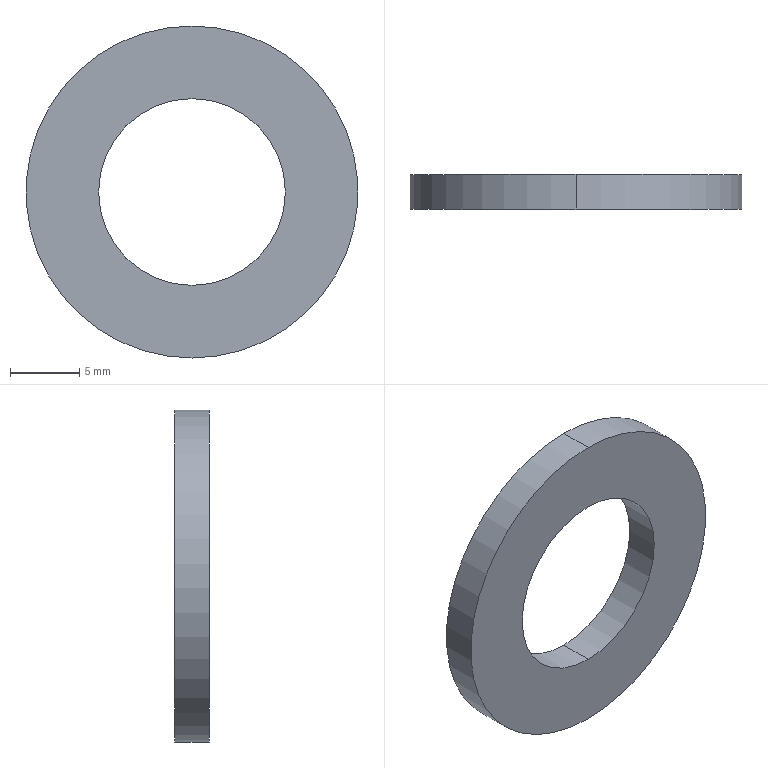Component | SolidWorks | GB_T95-2002[FlatWasherC-grade12]-1 | 1 solid | 6 faces | box 24 x 2.5 x 24 mm | volume 773 mm3 | cylinder 4 | plane 2 | commonest cylinder face diameters 24 x2 13.5 x2
build123d program:
from build123d import *

# Parameters (mm, degrees)
SKETCH1_W = 5.25
SKETCH1_H = 2.5


with BuildPart() as part:
    # Sketch1 → Base-Revolve (revolve)
    with BuildSketch(Plane.XY, mode=Mode.PRIVATE) as base_revolve_sk:
        with Locations((-9.375, 9.895)):
            Rectangle(SKETCH1_W, SKETCH1_H)
    revolve(base_revolve_sk.sketch.rotate(Axis((0, 0, 0), (0, 1, 0)), 270), axis=Axis((0, 0, 0), (0, 1, 0)))


solid = part.part

# Placed as in the assembly
solid = solid.moved(Location((96, 205.461, 0), (0, 0, 0)))
STEP:
#1=COLOUR_RGB('',0.7922,0.8196,0.9333);
#2=FILL_AREA_STYLE_COLOUR('',#1);
#3=FILL_AREA_STYLE('',(#2));
#4=SURFACE_STYLE_FILL_AREA(#3);
#5=SURFACE_SIDE_STYLE('',(#4));
#6=SURFACE_STYLE_USAGE(.BOTH.,#5);
#7=PRESENTATION_STYLE_ASSIGNMENT((#6));
#8=CARTESIAN_POINT('',(3.78,8.528,-0.4724));
#9=VERTEX_POINT('',#8);
#10=CARTESIAN_POINT('',(3.78,8.528,0.4724));
#11=VERTEX_POINT('',#10);
#12=CARTESIAN_POINT('',(3.78,8.528,0.));
#13=DIRECTION('',(0.,-1.,0.));
#14=DIRECTION('',(0.,0.,-1.));
#15=AXIS2_PLACEMENT_3D('',#12,#13,#14);
#16=CIRCLE('',#15,0.4724);
#17=EDGE_CURVE('',#9,#11,#16,.T.);
#18=ORIENTED_EDGE('',*,*,#17,.T.);
#19=CARTESIAN_POINT('',(3.78,8.429,0.4724));
#20=VERTEX_POINT('',#19);
#21=CARTESIAN_POINT('',(3.78,8.089,0.4724));
#22=DIRECTION('',(0.,-1.,0.));
#23=VECTOR('',#22,39.37);
#24=LINE('',#21,#23);
#25=EDGE_CURVE('',#11,#20,#24,.T.);
#26=ORIENTED_EDGE('',*,*,#25,.T.);
#27=CARTESIAN_POINT('',(3.78,8.429,-0.4724));
#28=VERTEX_POINT('',#27);
#29=CARTESIAN_POINT('',(3.78,8.429,0.));
#30=DIRECTION('',(0.,-1.,0.));
#31=DIRECTION('',(0.,0.,-1.));
#32=AXIS2_PLACEMENT_3D('',#29,#30,#31);
#33=CIRCLE('',#32,0.4724);
#34=EDGE_CURVE('',#28,#20,#33,.T.);
#35=ORIENTED_EDGE('',*,*,#34,.F.);
#36=CARTESIAN_POINT('',(3.78,8.089,-0.4724));
#37=DIRECTION('',(0.,-1.,0.));
#38=VECTOR('',#37,39.37);
#39=LINE('',#36,#38);
#40=EDGE_CURVE('',#9,#28,#39,.T.);
#41=ORIENTED_EDGE('',*,*,#40,.F.);
#42=EDGE_LOOP('',(#18,#26,#35,#41));
#43=FACE_OUTER_BOUND('',#42,.T.);
#44=CARTESIAN_POINT('',(3.78,8.089,0.));
#45=DIRECTION('',(0.,-1.,0.));
#46=DIRECTION('',(0.,0.,-1.));
#47=AXIS2_PLACEMENT_3D('',#44,#45,#46);
#48=CYLINDRICAL_SURFACE('',#47,0.4724);
#49=ADVANCED_FACE('',(#43),#48,.T.);
#50=CARTESIAN_POINT('',(3.78,8.528,0.2657));
#51=VERTEX_POINT('',#50);
#52=CARTESIAN_POINT('',(3.78,8.528,-0.2657));
#53=VERTEX_POINT('',#52);
#54=CARTESIAN_POINT('',(3.78,8.528,0.));
#55=DIRECTION('',(0.,-1.,0.));
#56=DIRECTION('',(0.,0.,-1.));
#57=AXIS2_PLACEMENT_3D('',#54,#55,#56);
#58=CIRCLE('',#57,0.2657);
#59=EDGE_CURVE('',#51,#53,#58,.T.);
#60=ORIENTED_EDGE('',*,*,#59,.F.);
#61=CARTESIAN_POINT('',(3.78,8.429,0.2657));
#62=VERTEX_POINT('',#61);
#63=CARTESIAN_POINT('',(3.78,8.089,0.2657));
#64=DIRECTION('',(0.,-1.,0.));
#65=VECTOR('',#64,39.37);
#66=LINE('',#63,#65);
#67=EDGE_CURVE('',#51,#62,#66,.T.);
#68=ORIENTED_EDGE('',*,*,#67,.T.);
#69=CARTESIAN_POINT('',(3.78,8.429,-0.2657));
#70=VERTEX_POINT('',#69);
#71=CARTESIAN_POINT('',(3.78,8.429,0.));
#72=DIRECTION('',(0.,-1.,0.));
#73=DIRECTION('',(0.,0.,-1.));
#74=AXIS2_PLACEMENT_3D('',#71,#72,#73);
#75=CIRCLE('',#74,0.2657);
#76=EDGE_CURVE('',#62,#70,#75,.T.);
#77=ORIENTED_EDGE('',*,*,#76,.T.);
#78=CARTESIAN_POINT('',(3.78,8.089,-0.2657));
#79=DIRECTION('',(0.,-1.,0.));
#80=VECTOR('',#79,39.37);
#81=LINE('',#78,#80);
#82=EDGE_CURVE('',#53,#70,#81,.T.);
#83=ORIENTED_EDGE('',*,*,#82,.F.);
#84=EDGE_LOOP('',(#60,#68,#77,#83));
#85=FACE_OUTER_BOUND('',#84,.T.);
#86=CARTESIAN_POINT('',(3.78,8.089,0.));
#87=DIRECTION('',(0.,-1.,0.));
#88=DIRECTION('',(0.,0.,-1.));
#89=AXIS2_PLACEMENT_3D('',#86,#87,#88);
#90=CYLINDRICAL_SURFACE('',#89,0.2657);
#91=ADVANCED_FACE('',(#85),#90,.F.);
#92=ORIENTED_EDGE('',*,*,#67,.F.);
#93=CARTESIAN_POINT('',(3.78,8.528,0.));
#94=DIRECTION('',(0.,-1.,0.));
#95=DIRECTION('',(0.,0.,-1.));
#96=AXIS2_PLACEMENT_3D('',#93,#94,#95);
#97=CIRCLE('',#96,0.2657);
#98=EDGE_CURVE('',#53,#51,#97,.T.);
#99=ORIENTED_EDGE('',*,*,#98,.F.);
#100=ORIENTED_EDGE('',*,*,#82,.T.);
#101=CARTESIAN_POINT('',(3.78,8.429,0.));
#102=DIRECTION('',(0.,-1.,0.));
#103=DIRECTION('',(0.,0.,-1.));
#104=AXIS2_PLACEMENT_3D('',#101,#102,#103);
#105=CIRCLE('',#104,0.2657);
#106=EDGE_CURVE('',#70,#62,#105,.T.);
#107=ORIENTED_EDGE('',*,*,#106,.T.);
#108=EDGE_LOOP('',(#92,#99,#100,#107));
#109=FACE_OUTER_BOUND('',#108,.T.);
#110=CARTESIAN_POINT('',(3.78,8.089,0.));
#111=DIRECTION('',(0.,-1.,0.));
#112=DIRECTION('',(0.,0.,-1.));
#113=AXIS2_PLACEMENT_3D('',#110,#111,#112);
#114=CYLINDRICAL_SURFACE('',#113,0.2657);
#115=ADVANCED_FACE('',(#109),#114,.F.);
#116=ORIENTED_EDGE('',*,*,#17,.F.);
#117=CARTESIAN_POINT('',(3.78,8.528,0.));
#118=DIRECTION('',(0.,-1.,0.));
#119=DIRECTION('',(0.,0.,-1.));
#120=AXIS2_PLACEMENT_3D('',#117,#118,#119);
#121=CIRCLE('',#120,0.4724);
#122=EDGE_CURVE('',#11,#9,#121,.T.);
#123=ORIENTED_EDGE('',*,*,#122,.F.);
#124=EDGE_LOOP('',(#116,#123));
#125=FACE_OUTER_BOUND('',#124,.T.);
#126=ORIENTED_EDGE('',*,*,#98,.T.);
#127=ORIENTED_EDGE('',*,*,#59,.T.);
#128=EDGE_LOOP('',(#126,#127));
#129=FACE_BOUND('',#128,.T.);
#130=CARTESIAN_POINT('',(3.514,8.528,0.));
#131=DIRECTION('',(0.,-1.,0.));
#132=DIRECTION('',(0.,0.,-1.));
#133=AXIS2_PLACEMENT_3D('',#130,#131,#132);
#134=PLANE('',#133);
#135=ADVANCED_FACE('',(#125,#129),#134,.F.);
#136=ORIENTED_EDGE('',*,*,#25,.F.);
#137=ORIENTED_EDGE('',*,*,#122,.T.);
#138=ORIENTED_EDGE('',*,*,#40,.T.);
#139=CARTESIAN_POINT('',(3.78,8.429,0.));
#140=DIRECTION('',(0.,-1.,0.));
#141=DIRECTION('',(0.,0.,-1.));
#142=AXIS2_PLACEMENT_3D('',#139,#140,#141);
#143=CIRCLE('',#142,0.4724);
#144=EDGE_CURVE('',#20,#28,#143,.T.);
#145=ORIENTED_EDGE('',*,*,#144,.F.);
#146=EDGE_LOOP('',(#136,#137,#138,#145));
#147=FACE_OUTER_BOUND('',#146,.T.);
#148=CARTESIAN_POINT('',(3.78,8.089,0.));
#149=DIRECTION('',(0.,-1.,0.));
#150=DIRECTION('',(0.,0.,-1.));
#151=AXIS2_PLACEMENT_3D('',#148,#149,#150);
#152=CYLINDRICAL_SURFACE('',#151,0.4724);
#153=ADVANCED_FACE('',(#147),#152,.T.);
#154=ORIENTED_EDGE('',*,*,#106,.F.);
#155=ORIENTED_EDGE('',*,*,#76,.F.);
#156=EDGE_LOOP('',(#154,#155));
#157=FACE_BOUND('',#156,.T.);
#158=ORIENTED_EDGE('',*,*,#34,.T.);
#159=ORIENTED_EDGE('',*,*,#144,.T.);
#160=EDGE_LOOP('',(#158,#159));
#161=FACE_OUTER_BOUND('',#160,.T.);
#162=CARTESIAN_POINT('',(3.514,8.429,0.));
#163=DIRECTION('',(0.,1.,0.));
#164=DIRECTION('',(0.,0.,1.));
#165=AXIS2_PLACEMENT_3D('',#162,#163,#164);
#166=PLANE('',#165);
#167=ADVANCED_FACE('',(#157,#161),#166,.F.);
#168=CLOSED_SHELL('',(#49,#91,#115,#135,#153,#167));
#169=MANIFOLD_SOLID_BREP('',#168);
#170=STYLED_ITEM('',(#7),#169);
#171=(LENGTH_UNIT()NAMED_UNIT(*)SI_UNIT($,.METRE.));
#172=LENGTH_MEASURE_WITH_UNIT(LENGTH_MEASURE(0.0254),#171);
#173=DIMENSIONAL_EXPONENTS(1.,0.,0.,0.,0.,0.,0.);
#174=(CONVERSION_BASED_UNIT('',#172)LENGTH_UNIT()NAMED_UNIT(#173));
#175=UNCERTAINTY_MEASURE_WITH_UNIT(LENGTH_MEASURE(0.00001),#174,'','');
#176=(NAMED_UNIT(*)PLANE_ANGLE_UNIT()SI_UNIT($,.RADIAN.));
#177=(NAMED_UNIT(*)SI_UNIT($,.STERADIAN.)SOLID_ANGLE_UNIT());
#178=(GEOMETRIC_REPRESENTATION_CONTEXT(3)GLOBAL_UNCERTAINTY_ASSIGNED_CONTEXT((#175))GLOBAL_UNIT_ASSIGNED_CONTEXT((#174,#176,#177))REPRESENTATION_CONTEXT('',''));
#179=MECHANICAL_DESIGN_GEOMETRIC_PRESENTATION_REPRESENTATION('',(#170),#178);
#180=PRESENTATION_LAYER_ASSIGNMENT('','',(#170));
#181=CARTESIAN_POINT('',(0.,0.,0.));
#182=DIRECTION('',(0.,0.,1.));
#183=DIRECTION('',(1.,0.,0.));
#184=AXIS2_PLACEMENT_3D('',#181,#182,#183);
#185=(LENGTH_UNIT()NAMED_UNIT(*)SI_UNIT($,.METRE.));
#186=LENGTH_MEASURE_WITH_UNIT(LENGTH_MEASURE(0.0254),#185);
#187=DIMENSIONAL_EXPONENTS(1.,0.,0.,0.,0.,0.,0.);
#188=(CONVERSION_BASED_UNIT('',#186)LENGTH_UNIT()NAMED_UNIT(#187));
#189=UNCERTAINTY_MEASURE_WITH_UNIT(LENGTH_MEASURE(0.00001),#188,'','');
#190=(NAMED_UNIT(*)PLANE_ANGLE_UNIT()SI_UNIT($,.RADIAN.));
#191=(NAMED_UNIT(*)SI_UNIT($,.STERADIAN.)SOLID_ANGLE_UNIT());
#192=(GEOMETRIC_REPRESENTATION_CONTEXT(3)GLOBAL_UNCERTAINTY_ASSIGNED_CONTEXT((#189))GLOBAL_UNIT_ASSIGNED_CONTEXT((#188,#190,#191))REPRESENTATION_CONTEXT('',''));
#193=ADVANCED_BREP_SHAPE_REPRESENTATION('',(#169,#184),#192);